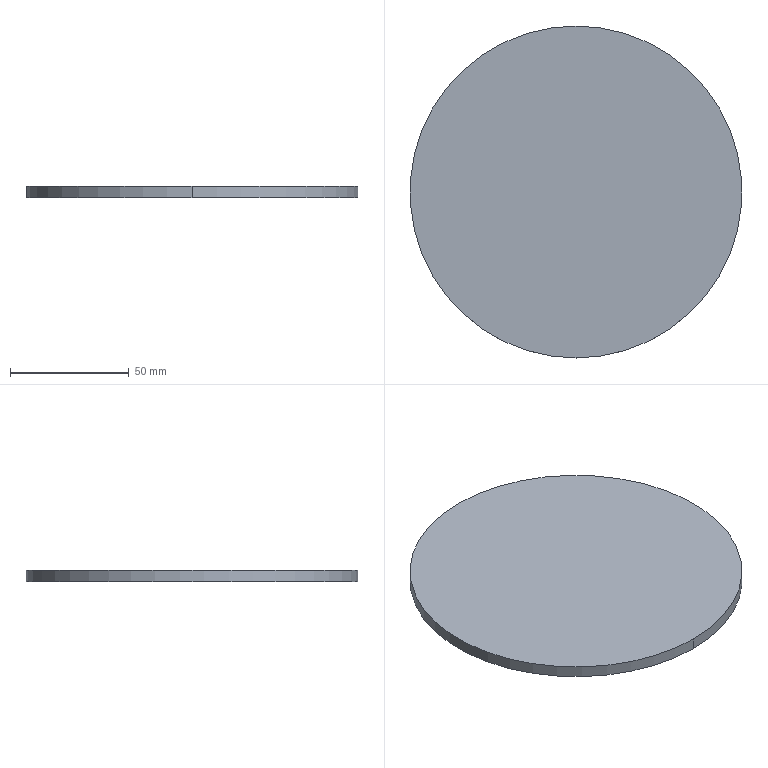Component | SolidWorks | Cap-1 | 1 solid | 4 faces | box 140 x 140 x 5 mm | volume 76969 mm3 | cylinder 2 | plane 2 | commonest cylinder face diameters 140 x2
build123d program:
from build123d import *

# Parameters (mm, degrees)
SKETCH1_R           = 70
BOSS_EXTRUDE1_DEPTH = 5


with BuildPart() as part:
    # Sketch1 → Boss-Extrude1 (new body)
    with BuildSketch(Plane(origin=(0, 0, 0), x_dir=(1, 0, 0), z_dir=(0, 1, 0))):
        with Locations(Location((0, 0, 0), (0, 0, 270))):
            Circle(SKETCH1_R)
    extrude(amount=BOSS_EXTRUDE1_DEPTH)


solid = part.part

# Placed as in the assembly
solid = solid.moved(Location((-99.458, -18.912, 1056.75), (90, 0, 0)))
STEP:
#1=COLOUR_RGB('',0.7922,0.8196,0.9333);
#2=FILL_AREA_STYLE_COLOUR('',#1);
#3=FILL_AREA_STYLE('',(#2));
#4=SURFACE_STYLE_FILL_AREA(#3);
#5=SURFACE_SIDE_STYLE('',(#4));
#6=SURFACE_STYLE_USAGE(.BOTH.,#5);
#7=PRESENTATION_STYLE_ASSIGNMENT((#6));
#8=CARTESIAN_POINT('',(-3.916,-3.5,41.801));
#9=VERTEX_POINT('',#8);
#10=CARTESIAN_POINT('',(-3.916,2.011,41.801));
#11=VERTEX_POINT('',#10);
#12=CARTESIAN_POINT('',(-3.916,-0.7446,41.801));
#13=DIRECTION('',(0.,0.,1.));
#14=DIRECTION('',(0.,-1.,0.));
#15=AXIS2_PLACEMENT_3D('',#12,#13,#14);
#16=CIRCLE('',#15,2.756);
#17=EDGE_CURVE('',#9,#11,#16,.T.);
#18=ORIENTED_EDGE('',*,*,#17,.F.);
#19=CARTESIAN_POINT('',(-3.916,-3.5,41.604));
#20=VERTEX_POINT('',#19);
#21=CARTESIAN_POINT('',(-3.916,-3.5,41.801));
#22=DIRECTION('',(0.,0.,-1.));
#23=VECTOR('',#22,39.37);
#24=LINE('',#21,#23);
#25=EDGE_CURVE('',#9,#20,#24,.T.);
#26=ORIENTED_EDGE('',*,*,#25,.T.);
#27=CARTESIAN_POINT('',(-3.916,2.011,41.604));
#28=VERTEX_POINT('',#27);
#29=CARTESIAN_POINT('',(-3.916,-0.7446,41.604));
#30=DIRECTION('',(0.,0.,1.));
#31=DIRECTION('',(0.,-1.,0.));
#32=AXIS2_PLACEMENT_3D('',#29,#30,#31);
#33=CIRCLE('',#32,2.756);
#34=EDGE_CURVE('',#20,#28,#33,.T.);
#35=ORIENTED_EDGE('',*,*,#34,.T.);
#36=CARTESIAN_POINT('',(-3.916,2.011,41.801));
#37=DIRECTION('',(0.,0.,-1.));
#38=VECTOR('',#37,39.37);
#39=LINE('',#36,#38);
#40=EDGE_CURVE('',#11,#28,#39,.T.);
#41=ORIENTED_EDGE('',*,*,#40,.F.);
#42=EDGE_LOOP('',(#18,#26,#35,#41));
#43=FACE_OUTER_BOUND('',#42,.T.);
#44=CARTESIAN_POINT('',(-3.916,-0.7446,41.801));
#45=DIRECTION('',(0.,0.,-1.));
#46=DIRECTION('',(0.,1.,0.));
#47=AXIS2_PLACEMENT_3D('',#44,#45,#46);
#48=CYLINDRICAL_SURFACE('',#47,2.756);
#49=ADVANCED_FACE('',(#43),#48,.T.);
#50=ORIENTED_EDGE('',*,*,#25,.F.);
#51=CARTESIAN_POINT('',(-3.916,-0.7446,41.801));
#52=DIRECTION('',(0.,0.,1.));
#53=DIRECTION('',(0.,-1.,0.));
#54=AXIS2_PLACEMENT_3D('',#51,#52,#53);
#55=CIRCLE('',#54,2.756);
#56=EDGE_CURVE('',#11,#9,#55,.T.);
#57=ORIENTED_EDGE('',*,*,#56,.F.);
#58=ORIENTED_EDGE('',*,*,#40,.T.);
#59=CARTESIAN_POINT('',(-3.916,-0.7446,41.604));
#60=DIRECTION('',(0.,0.,1.));
#61=DIRECTION('',(0.,-1.,0.));
#62=AXIS2_PLACEMENT_3D('',#59,#60,#61);
#63=CIRCLE('',#62,2.756);
#64=EDGE_CURVE('',#28,#20,#63,.T.);
#65=ORIENTED_EDGE('',*,*,#64,.T.);
#66=EDGE_LOOP('',(#50,#57,#58,#65));
#67=FACE_OUTER_BOUND('',#66,.T.);
#68=CARTESIAN_POINT('',(-3.916,-0.7446,41.801));
#69=DIRECTION('',(0.,0.,-1.));
#70=DIRECTION('',(0.,1.,0.));
#71=AXIS2_PLACEMENT_3D('',#68,#69,#70);
#72=CYLINDRICAL_SURFACE('',#71,2.756);
#73=ADVANCED_FACE('',(#67),#72,.T.);
#74=ORIENTED_EDGE('',*,*,#56,.T.);
#75=ORIENTED_EDGE('',*,*,#17,.T.);
#76=EDGE_LOOP('',(#74,#75));
#77=FACE_OUTER_BOUND('',#76,.T.);
#78=CARTESIAN_POINT('',(-3.916,-0.7446,41.801));
#79=DIRECTION('',(0.,0.,1.));
#80=DIRECTION('',(0.,-1.,0.));
#81=AXIS2_PLACEMENT_3D('',#78,#79,#80);
#82=PLANE('',#81);
#83=ADVANCED_FACE('',(#77),#82,.T.);
#84=ORIENTED_EDGE('',*,*,#64,.F.);
#85=ORIENTED_EDGE('',*,*,#34,.F.);
#86=EDGE_LOOP('',(#84,#85));
#87=FACE_OUTER_BOUND('',#86,.T.);
#88=CARTESIAN_POINT('',(-3.916,-0.7446,41.604));
#89=DIRECTION('',(0.,0.,1.));
#90=DIRECTION('',(0.,-1.,0.));
#91=AXIS2_PLACEMENT_3D('',#88,#89,#90);
#92=PLANE('',#91);
#93=ADVANCED_FACE('',(#87),#92,.F.);
#94=CLOSED_SHELL('',(#49,#73,#83,#93));
#95=MANIFOLD_SOLID_BREP('',#94);
#96=STYLED_ITEM('',(#7),#95);
#97=(LENGTH_UNIT()NAMED_UNIT(*)SI_UNIT($,.METRE.));
#98=LENGTH_MEASURE_WITH_UNIT(LENGTH_MEASURE(0.0254),#97);
#99=DIMENSIONAL_EXPONENTS(1.,0.,0.,0.,0.,0.,0.);
#100=(CONVERSION_BASED_UNIT('',#98)LENGTH_UNIT()NAMED_UNIT(#99));
#101=UNCERTAINTY_MEASURE_WITH_UNIT(LENGTH_MEASURE(0.00001),#100,'','');
#102=(NAMED_UNIT(*)PLANE_ANGLE_UNIT()SI_UNIT($,.RADIAN.));
#103=(NAMED_UNIT(*)SI_UNIT($,.STERADIAN.)SOLID_ANGLE_UNIT());
#104=(GEOMETRIC_REPRESENTATION_CONTEXT(3)GLOBAL_UNCERTAINTY_ASSIGNED_CONTEXT((#101))GLOBAL_UNIT_ASSIGNED_CONTEXT((#100,#102,#103))REPRESENTATION_CONTEXT('',''));
#105=MECHANICAL_DESIGN_GEOMETRIC_PRESENTATION_REPRESENTATION('',(#96),#104);
#106=CARTESIAN_POINT('',(0.,0.,0.));
#107=DIRECTION('',(0.,0.,1.));
#108=DIRECTION('',(1.,0.,0.));
#109=AXIS2_PLACEMENT_3D('',#106,#107,#108);
#110=(LENGTH_UNIT()NAMED_UNIT(*)SI_UNIT($,.METRE.));
#111=LENGTH_MEASURE_WITH_UNIT(LENGTH_MEASURE(0.0254),#110);
#112=DIMENSIONAL_EXPONENTS(1.,0.,0.,0.,0.,0.,0.);
#113=(CONVERSION_BASED_UNIT('',#111)LENGTH_UNIT()NAMED_UNIT(#112));
#114=UNCERTAINTY_MEASURE_WITH_UNIT(LENGTH_MEASURE(0.00001),#113,'','');
#115=(NAMED_UNIT(*)PLANE_ANGLE_UNIT()SI_UNIT($,.RADIAN.));
#116=(NAMED_UNIT(*)SI_UNIT($,.STERADIAN.)SOLID_ANGLE_UNIT());
#117=(GEOMETRIC_REPRESENTATION_CONTEXT(3)GLOBAL_UNCERTAINTY_ASSIGNED_CONTEXT((#114))GLOBAL_UNIT_ASSIGNED_CONTEXT((#113,#115,#116))REPRESENTATION_CONTEXT('',''));
#118=ADVANCED_BREP_SHAPE_REPRESENTATION('',(#95,#109),#117);
#119=PRESENTATION_LAYER_ASSIGNMENT('','',(#96));